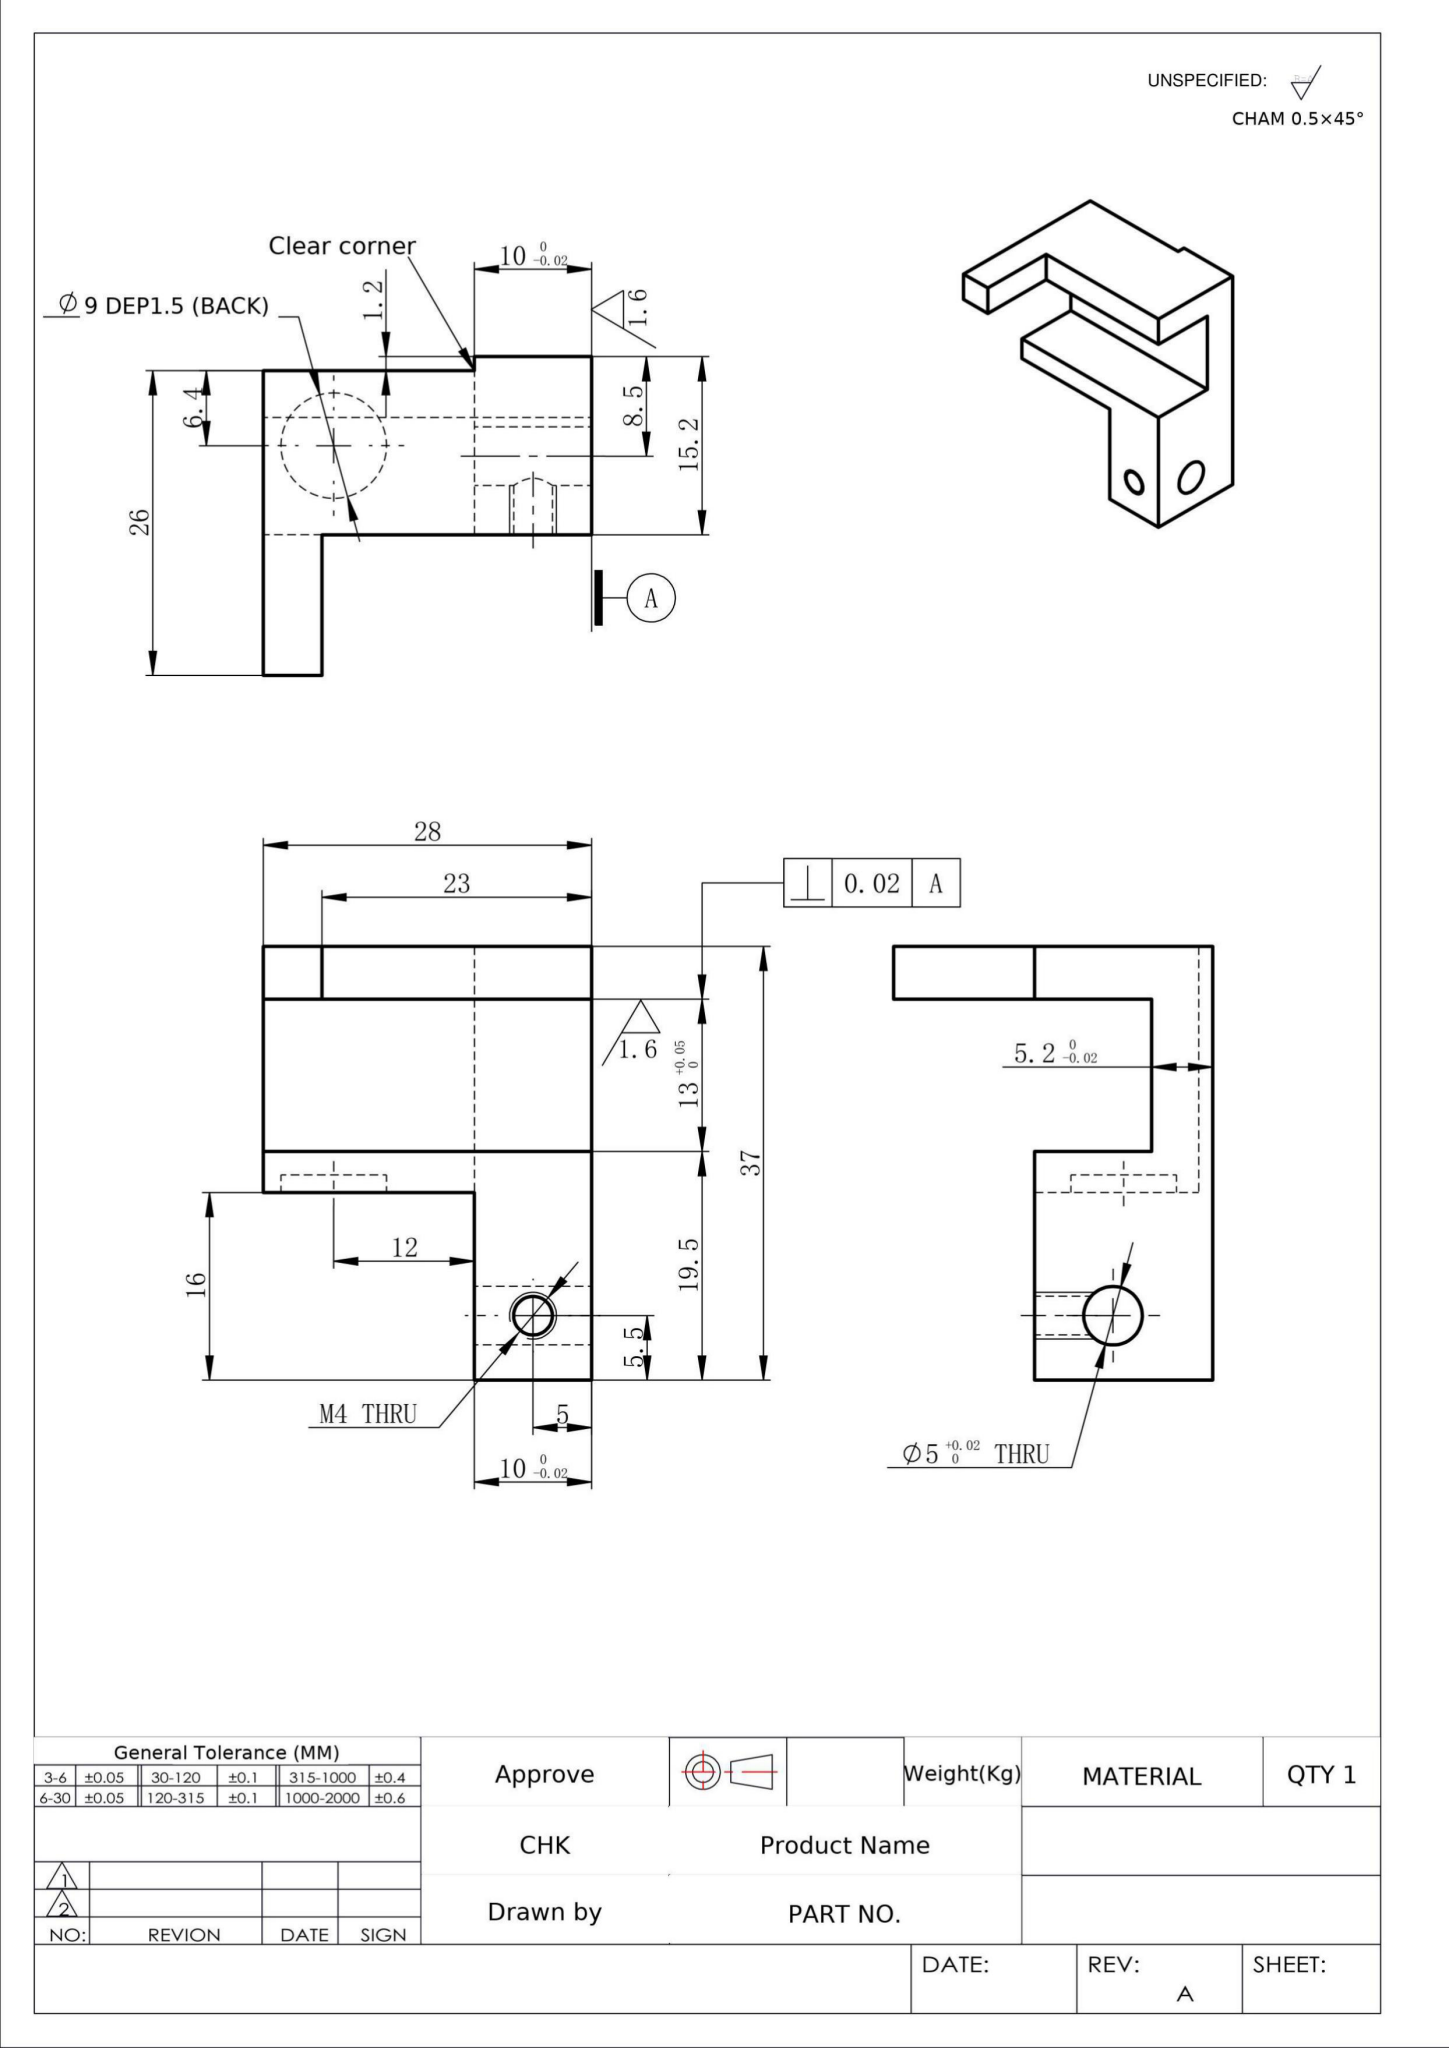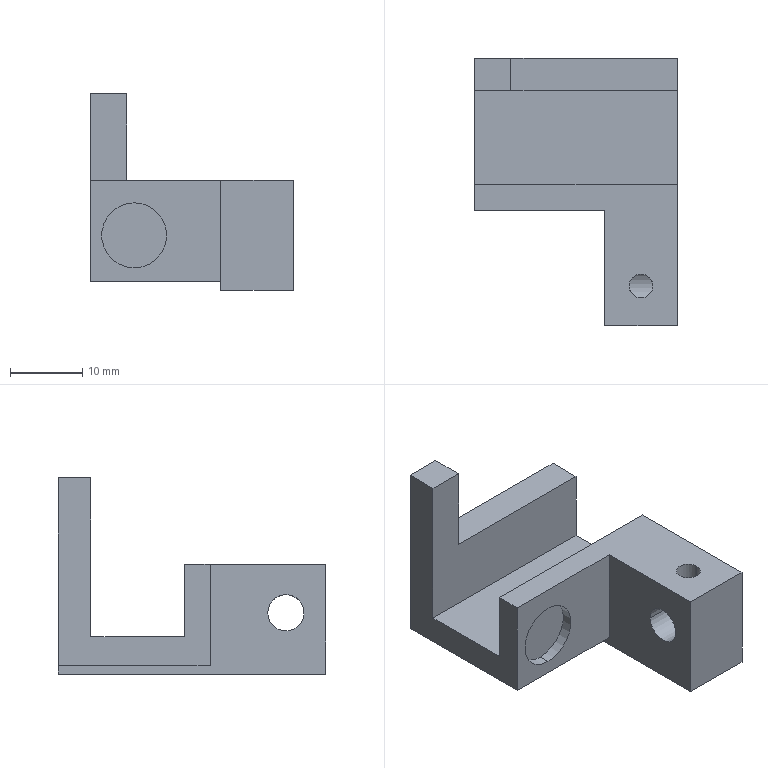Part | NX | mm | Offset Slide Clamp Block | 1 solid | 22 faces | box 28 x 37 x 27.2 mm | volume 7217 mm3 | plane 16 | cylinder 6 | commonest cylinder face diameters 3.3 x2 5 x2 9 x2
STEP:
#1=COLOUR_RGB('',0.7961,0.8235,0.9373);
#2=FILL_AREA_STYLE_COLOUR('',#1);
#3=FILL_AREA_STYLE('',(#2));
#4=SURFACE_STYLE_FILL_AREA(#3);
#5=SURFACE_SIDE_STYLE('',(#4));
#6=SURFACE_STYLE_USAGE(.BOTH.,#5);
#7=PRESENTATION_STYLE_ASSIGNMENT((#6));
#8=CARTESIAN_POINT('',(-6.65,-31.5,11.));
#9=VERTEX_POINT('',#8);
#10=CARTESIAN_POINT('',(-3.35,-31.5,11.));
#11=VERTEX_POINT('',#10);
#12=CARTESIAN_POINT('',(-6.65,-31.5,11.));
#13=CARTESIAN_POINT('',(-6.65,-31.611,11.));
#14=CARTESIAN_POINT('',(-6.639,-31.724,10.992));
#15=CARTESIAN_POINT('',(-6.594,-31.941,10.963));
#16=CARTESIAN_POINT('',(-6.561,-32.045,10.942));
#17=CARTESIAN_POINT('',(-6.433,-32.346,10.862));
#18=CARTESIAN_POINT('',(-6.311,-32.524,10.787));
#19=CARTESIAN_POINT('',(-6.088,-32.745,10.67));
#20=CARTESIAN_POINT('',(-6.008,-32.811,10.63));
#21=CARTESIAN_POINT('',(-5.834,-32.928,10.553));
#22=CARTESIAN_POINT('',(-5.74,-32.979,10.516));
#23=CARTESIAN_POINT('',(-5.445,-33.103,10.421));
#24=CARTESIAN_POINT('',(-5.224,-33.15,10.378));
#25=CARTESIAN_POINT('',(-4.775,-33.15,10.378));
#26=CARTESIAN_POINT('',(-4.553,-33.102,10.422));
#27=CARTESIAN_POINT('',(-4.16,-32.936,10.549));
#28=CARTESIAN_POINT('',(-3.984,-32.816,10.632));
#29=CARTESIAN_POINT('',(-3.688,-32.522,10.788));
#30=CARTESIAN_POINT('',(-3.566,-32.344,10.862));
#31=CARTESIAN_POINT('',(-3.44,-32.047,10.942));
#32=CARTESIAN_POINT('',(-3.406,-31.941,10.963));
#33=CARTESIAN_POINT('',(-3.361,-31.724,10.992));
#34=CARTESIAN_POINT('',(-3.35,-31.613,11.));
#35=CARTESIAN_POINT('',(-3.35,-31.5,11.));
#36=B_SPLINE_CURVE_WITH_KNOTS('',3,(#12,#13,#14,#15,#16,#17,#18,#19,#20,#21,#22,#23,#24,#25,#26,#27,#28,#29,#30,#31,#32,#33,#34,#35),.UNSPECIFIED.,.F.,.F.,(4,2,2,2,2,2,2,2,2,2,2,4),(0.005328,0.005661,0.005993,0.006658,0.006991,0.007324,0.007989,0.008654,0.009319,0.009984,0.01032,0.01065),.UNSPECIFIED.);
#37=EDGE_CURVE('',#9,#11,#36,.T.);
#38=ORIENTED_EDGE('',*,*,#37,.F.);
#39=CARTESIAN_POINT('',(-6.65,-31.5,15.2));
#40=VERTEX_POINT('',#39);
#41=CARTESIAN_POINT('',(-6.65,-31.5,15.2));
#42=DIRECTION('',(0.,0.,1.));
#43=VECTOR('',#42,1000.);
#44=LINE('',#41,#43);
#45=EDGE_CURVE('',#9,#40,#44,.T.);
#46=ORIENTED_EDGE('',*,*,#45,.T.);
#47=CARTESIAN_POINT('',(-3.35,-31.5,15.2));
#48=VERTEX_POINT('',#47);
#49=CARTESIAN_POINT('',(-5.,-31.5,15.2));
#50=DIRECTION('',(0.,0.,1.));
#51=DIRECTION('',(1.,0.,0.));
#52=AXIS2_PLACEMENT_3D('',#49,#50,#51);
#53=CIRCLE('',#52,1.65);
#54=EDGE_CURVE('',#40,#48,#53,.T.);
#55=ORIENTED_EDGE('',*,*,#54,.T.);
#56=CARTESIAN_POINT('',(-3.35,-31.5,15.2));
#57=DIRECTION('',(0.,0.,1.));
#58=VECTOR('',#57,1000.);
#59=LINE('',#56,#58);
#60=EDGE_CURVE('',#11,#48,#59,.T.);
#61=ORIENTED_EDGE('',*,*,#60,.F.);
#62=EDGE_LOOP('',(#38,#46,#55,#61));
#63=FACE_OUTER_BOUND('',#62,.T.);
#64=CARTESIAN_POINT('',(-5.,-31.5,15.2));
#65=DIRECTION('',(0.,0.,1.));
#66=DIRECTION('',(1.,0.,0.));
#67=AXIS2_PLACEMENT_3D('',#64,#65,#66);
#68=CYLINDRICAL_SURFACE('',#67,1.65);
#69=ADVANCED_FACE('',(#63),#68,.F.);
#70=CARTESIAN_POINT('',(-10.,-34.,8.5));
#71=VERTEX_POINT('',#70);
#72=CARTESIAN_POINT('',(-10.,-29.,8.5));
#73=VERTEX_POINT('',#72);
#74=CARTESIAN_POINT('',(-10.,-31.5,8.5));
#75=DIRECTION('',(1.,0.,0.));
#76=DIRECTION('',(0.,1.,0.));
#77=AXIS2_PLACEMENT_3D('',#74,#75,#76);
#78=CIRCLE('',#77,2.5);
#79=EDGE_CURVE('',#71,#73,#78,.T.);
#80=ORIENTED_EDGE('',*,*,#79,.F.);
#81=CARTESIAN_POINT('',(0.,-34.,8.5));
#82=VERTEX_POINT('',#81);
#83=CARTESIAN_POINT('',(-28.,-34.,8.5));
#84=DIRECTION('',(1.,0.,0.));
#85=VECTOR('',#84,1000.);
#86=LINE('',#83,#85);
#87=EDGE_CURVE('',#71,#82,#86,.T.);
#88=ORIENTED_EDGE('',*,*,#87,.T.);
#89=CARTESIAN_POINT('',(0.,-29.,8.5));
#90=VERTEX_POINT('',#89);
#91=CARTESIAN_POINT('',(0.,-31.5,8.5));
#92=DIRECTION('',(1.,0.,0.));
#93=DIRECTION('',(-0.,1.,0.));
#94=AXIS2_PLACEMENT_3D('',#91,#92,#93);
#95=CIRCLE('',#94,2.5);
#96=EDGE_CURVE('',#82,#90,#95,.T.);
#97=ORIENTED_EDGE('',*,*,#96,.T.);
#98=CARTESIAN_POINT('',(-28.,-29.,8.5));
#99=DIRECTION('',(1.,0.,0.));
#100=VECTOR('',#99,1000.);
#101=LINE('',#98,#100);
#102=EDGE_CURVE('',#73,#90,#101,.T.);
#103=ORIENTED_EDGE('',*,*,#102,.F.);
#104=EDGE_LOOP('',(#80,#88,#97,#103));
#105=FACE_OUTER_BOUND('',#104,.T.);
#106=CARTESIAN_POINT('',(-28.,-31.5,8.5));
#107=DIRECTION('',(1.,0.,0.));
#108=DIRECTION('',(0.,1.,0.));
#109=AXIS2_PLACEMENT_3D('',#106,#107,#108);
#110=CYLINDRICAL_SURFACE('',#109,2.5);
#111=ADVANCED_FACE('',(#105),#110,.F.);
#112=CARTESIAN_POINT('',(-22.,-19.5,12.1));
#113=VERTEX_POINT('',#112);
#114=CARTESIAN_POINT('',(-22.,-19.5,3.1));
#115=VERTEX_POINT('',#114);
#116=CARTESIAN_POINT('',(-22.,-19.5,7.6));
#117=DIRECTION('',(0.,-1.,0.));
#118=DIRECTION('',(0.,0.,-1.));
#119=AXIS2_PLACEMENT_3D('',#116,#117,#118);
#120=CIRCLE('',#119,4.5);
#121=EDGE_CURVE('',#113,#115,#120,.T.);
#122=ORIENTED_EDGE('',*,*,#121,.F.);
#123=CARTESIAN_POINT('',(-22.,-21.,12.1));
#124=VERTEX_POINT('',#123);
#125=CARTESIAN_POINT('',(-22.,-19.5,12.1));
#126=DIRECTION('',(0.,-1.,0.));
#127=VECTOR('',#126,1000.);
#128=LINE('',#125,#127);
#129=EDGE_CURVE('',#113,#124,#128,.T.);
#130=ORIENTED_EDGE('',*,*,#129,.T.);
#131=CARTESIAN_POINT('',(-22.,-21.,3.1));
#132=VERTEX_POINT('',#131);
#133=CARTESIAN_POINT('',(-22.,-21.,7.6));
#134=DIRECTION('',(0.,-1.,0.));
#135=DIRECTION('',(0.,0.,-1.));
#136=AXIS2_PLACEMENT_3D('',#133,#134,#135);
#137=CIRCLE('',#136,4.5);
#138=EDGE_CURVE('',#124,#132,#137,.T.);
#139=ORIENTED_EDGE('',*,*,#138,.T.);
#140=CARTESIAN_POINT('',(-22.,-19.5,3.1));
#141=DIRECTION('',(0.,-1.,0.));
#142=VECTOR('',#141,1000.);
#143=LINE('',#140,#142);
#144=EDGE_CURVE('',#115,#132,#143,.T.);
#145=ORIENTED_EDGE('',*,*,#144,.F.);
#146=EDGE_LOOP('',(#122,#130,#139,#145));
#147=FACE_OUTER_BOUND('',#146,.T.);
#148=CARTESIAN_POINT('',(-22.,-19.5,7.6));
#149=DIRECTION('',(0.,-1.,0.));
#150=DIRECTION('',(0.,0.,-1.));
#151=AXIS2_PLACEMENT_3D('',#148,#149,#150);
#152=CYLINDRICAL_SURFACE('',#151,4.5);
#153=ADVANCED_FACE('',(#147),#152,.F.);
#154=CARTESIAN_POINT('',(-23.,0.,15.2));
#155=VERTEX_POINT('',#154);
#156=CARTESIAN_POINT('',(-23.,-4.5,15.2));
#157=VERTEX_POINT('',#156);
#158=CARTESIAN_POINT('',(-23.,-4.5,15.2));
#159=DIRECTION('',(0.,-1.,0.));
#160=VECTOR('',#159,1000.);
#161=LINE('',#158,#160);
#162=EDGE_CURVE('',#155,#157,#161,.T.);
#163=ORIENTED_EDGE('',*,*,#162,.T.);
#164=CARTESIAN_POINT('',(0.,-4.5,15.2));
#165=VERTEX_POINT('',#164);
#166=CARTESIAN_POINT('',(-28.,-4.5,15.2));
#167=DIRECTION('',(-1.,0.,0.));
#168=VECTOR('',#167,1000.);
#169=LINE('',#166,#168);
#170=EDGE_CURVE('',#165,#157,#169,.T.);
#171=ORIENTED_EDGE('',*,*,#170,.F.);
#172=CARTESIAN_POINT('',(0.,0.,15.2));
#173=VERTEX_POINT('',#172);
#174=CARTESIAN_POINT('',(0.,0.,15.2));
#175=DIRECTION('',(-0.,1.,0.));
#176=VECTOR('',#175,1000.);
#177=LINE('',#174,#176);
#178=EDGE_CURVE('',#165,#173,#177,.T.);
#179=ORIENTED_EDGE('',*,*,#178,.T.);
#180=CARTESIAN_POINT('',(-23.,0.,15.2));
#181=DIRECTION('',(-1.,0.,0.));
#182=VECTOR('',#181,1000.);
#183=LINE('',#180,#182);
#184=EDGE_CURVE('',#173,#155,#183,.T.);
#185=ORIENTED_EDGE('',*,*,#184,.T.);
#186=EDGE_LOOP('',(#163,#171,#179,#185));
#187=FACE_OUTER_BOUND('',#186,.T.);
#188=CARTESIAN_POINT('',(-28.,-4.5,15.2));
#189=DIRECTION('',(0.,0.,-1.));
#190=DIRECTION('',(-1.,0.,0.));
#191=AXIS2_PLACEMENT_3D('',#188,#189,#190);
#192=PLANE('',#191);
#193=ADVANCED_FACE('',(#187),#192,.F.);
#194=CARTESIAN_POINT('',(0.,-31.5,8.5));
#195=DIRECTION('',(1.,0.,0.));
#196=DIRECTION('',(-0.,1.,0.));
#197=AXIS2_PLACEMENT_3D('',#194,#195,#196);
#198=CIRCLE('',#197,2.5);
#199=EDGE_CURVE('',#90,#82,#198,.T.);
#200=ORIENTED_EDGE('',*,*,#199,.F.);
#201=ORIENTED_EDGE('',*,*,#96,.F.);
#202=EDGE_LOOP('',(#200,#201));
#203=FACE_BOUND('',#202,.T.);
#204=ORIENTED_EDGE('',*,*,#178,.F.);
#205=CARTESIAN_POINT('',(0.,-4.5,5.2));
#206=VERTEX_POINT('',#205);
#207=CARTESIAN_POINT('',(0.,-4.5,5.2));
#208=DIRECTION('',(0.,0.,1.));
#209=VECTOR('',#208,1000.);
#210=LINE('',#207,#209);
#211=EDGE_CURVE('',#206,#165,#210,.T.);
#212=ORIENTED_EDGE('',*,*,#211,.F.);
#213=CARTESIAN_POINT('',(0.,-17.5,5.2));
#214=VERTEX_POINT('',#213);
#215=CARTESIAN_POINT('',(0.,-4.5,5.2));
#216=DIRECTION('',(-0.,1.,0.));
#217=VECTOR('',#216,1000.);
#218=LINE('',#215,#217);
#219=EDGE_CURVE('',#214,#206,#218,.T.);
#220=ORIENTED_EDGE('',*,*,#219,.F.);
#221=CARTESIAN_POINT('',(0.,-17.5,15.2));
#222=VERTEX_POINT('',#221);
#223=CARTESIAN_POINT('',(0.,-17.5,5.2));
#224=DIRECTION('',(0.,0.,1.));
#225=VECTOR('',#224,1000.);
#226=LINE('',#223,#225);
#227=EDGE_CURVE('',#214,#222,#226,.T.);
#228=ORIENTED_EDGE('',*,*,#227,.T.);
#229=CARTESIAN_POINT('',(0.,-37.,15.2));
#230=VERTEX_POINT('',#229);
#231=CARTESIAN_POINT('',(0.,0.,15.2));
#232=DIRECTION('',(-0.,1.,0.));
#233=VECTOR('',#232,1000.);
#234=LINE('',#231,#233);
#235=EDGE_CURVE('',#230,#222,#234,.T.);
#236=ORIENTED_EDGE('',*,*,#235,.F.);
#237=CARTESIAN_POINT('',(0.,-37.,0.));
#238=VERTEX_POINT('',#237);
#239=CARTESIAN_POINT('',(0.,-37.,27.2));
#240=DIRECTION('',(0.,0.,-1.));
#241=VECTOR('',#240,1000.);
#242=LINE('',#239,#241);
#243=EDGE_CURVE('',#230,#238,#242,.T.);
#244=ORIENTED_EDGE('',*,*,#243,.T.);
#245=CARTESIAN_POINT('',(0.,0.,0.));
#246=VERTEX_POINT('',#245);
#247=CARTESIAN_POINT('',(0.,0.,0.));
#248=DIRECTION('',(-0.,1.,0.));
#249=VECTOR('',#248,1000.);
#250=LINE('',#247,#249);
#251=EDGE_CURVE('',#238,#246,#250,.T.);
#252=ORIENTED_EDGE('',*,*,#251,.T.);
#253=CARTESIAN_POINT('',(0.,0.,27.2));
#254=DIRECTION('',(0.,0.,-1.));
#255=VECTOR('',#254,1000.);
#256=LINE('',#253,#255);
#257=EDGE_CURVE('',#173,#246,#256,.T.);
#258=ORIENTED_EDGE('',*,*,#257,.F.);
#259=EDGE_LOOP('',(#204,#212,#220,#228,#236,#244,#252,#258));
#260=FACE_OUTER_BOUND('',#259,.T.);
#261=CARTESIAN_POINT('',(0.,0.,27.2));
#262=DIRECTION('',(-1.,-0.,0.));
#263=DIRECTION('',(0.,-1.,0.));
#264=AXIS2_PLACEMENT_3D('',#261,#262,#263);
#265=PLANE('',#264);
#266=ADVANCED_FACE('',(#203,#260),#265,.F.);
#267=CARTESIAN_POINT('',(-10.,-0.,0.));
#268=VERTEX_POINT('',#267);
#269=CARTESIAN_POINT('',(0.,0.,0.));
#270=DIRECTION('',(-1.,-0.,0.));
#271=VECTOR('',#270,1000.);
#272=LINE('',#269,#271);
#273=EDGE_CURVE('',#246,#268,#272,.T.);
#274=ORIENTED_EDGE('',*,*,#273,.T.);
#275=CARTESIAN_POINT('',(-10.,-0.,1.2));
#276=VERTEX_POINT('',#275);
#277=CARTESIAN_POINT('',(-10.,-0.,1.2));
#278=DIRECTION('',(0.,0.,-1.));
#279=VECTOR('',#278,1000.);
#280=LINE('',#277,#279);
#281=EDGE_CURVE('',#276,#268,#280,.T.);
#282=ORIENTED_EDGE('',*,*,#281,.F.);
#283=CARTESIAN_POINT('',(-28.,-0.,1.2));
#284=VERTEX_POINT('',#283);
#285=CARTESIAN_POINT('',(-10.,-0.,1.2));
#286=DIRECTION('',(1.,0.,0.));
#287=VECTOR('',#286,1000.);
#288=LINE('',#285,#287);
#289=EDGE_CURVE('',#284,#276,#288,.T.);
#290=ORIENTED_EDGE('',*,*,#289,.F.);
#291=CARTESIAN_POINT('',(-28.,-0.,27.2));
#292=VERTEX_POINT('',#291);
#293=CARTESIAN_POINT('',(-28.,-0.,27.2));
#294=DIRECTION('',(0.,0.,-1.));
#295=VECTOR('',#294,1000.);
#296=LINE('',#293,#295);
#297=EDGE_CURVE('',#292,#284,#296,.T.);
#298=ORIENTED_EDGE('',*,*,#297,.F.);
#299=CARTESIAN_POINT('',(-23.,-0.,27.2));
#300=VERTEX_POINT('',#299);
#301=CARTESIAN_POINT('',(0.,0.,27.2));
#302=DIRECTION('',(-1.,-0.,0.));
#303=VECTOR('',#302,1000.);
#304=LINE('',#301,#303);
#305=EDGE_CURVE('',#300,#292,#304,.T.);
#306=ORIENTED_EDGE('',*,*,#305,.F.);
#307=CARTESIAN_POINT('',(-23.,0.,15.2));
#308=DIRECTION('',(0.,0.,1.));
#309=VECTOR('',#308,1000.);
#310=LINE('',#307,#309);
#311=EDGE_CURVE('',#155,#300,#310,.T.);
#312=ORIENTED_EDGE('',*,*,#311,.F.);
#313=ORIENTED_EDGE('',*,*,#184,.F.);
#314=ORIENTED_EDGE('',*,*,#257,.T.);
#315=EDGE_LOOP('',(#274,#282,#290,#298,#306,#312,#313,#314));
#316=FACE_OUTER_BOUND('',#315,.T.);
#317=CARTESIAN_POINT('',(0.,0.,27.2));
#318=DIRECTION('',(0.,-1.,0.));
#319=DIRECTION('',(1.,0.,0.));
#320=AXIS2_PLACEMENT_3D('',#317,#318,#319);
#321=PLANE('',#320);
#322=ADVANCED_FACE('',(#316),#321,.F.);
#323=ORIENTED_EDGE('',*,*,#297,.T.);
#324=CARTESIAN_POINT('',(-28.,-21.,1.2));
#325=VERTEX_POINT('',#324);
#326=CARTESIAN_POINT('',(-28.,-21.,1.2));
#327=DIRECTION('',(0.,1.,0.));
#328=VECTOR('',#327,1000.);
#329=LINE('',#326,#328);
#330=EDGE_CURVE('',#325,#284,#329,.T.);
#331=ORIENTED_EDGE('',*,*,#330,.F.);
#332=CARTESIAN_POINT('',(-28.,-21.,15.2));
#333=VERTEX_POINT('',#332);
#334=CARTESIAN_POINT('',(-28.,-21.,27.2));
#335=DIRECTION('',(0.,0.,-1.));
#336=VECTOR('',#335,1000.);
#337=LINE('',#334,#336);
#338=EDGE_CURVE('',#333,#325,#337,.T.);
#339=ORIENTED_EDGE('',*,*,#338,.F.);
#340=CARTESIAN_POINT('',(-28.,-17.5,15.2));
#341=VERTEX_POINT('',#340);
#342=CARTESIAN_POINT('',(-28.,-21.,15.2));
#343=DIRECTION('',(0.,-1.,0.));
#344=VECTOR('',#343,1000.);
#345=LINE('',#342,#344);
#346=EDGE_CURVE('',#341,#333,#345,.T.);
#347=ORIENTED_EDGE('',*,*,#346,.F.);
#348=CARTESIAN_POINT('',(-28.,-17.5,5.2));
#349=VERTEX_POINT('',#348);
#350=CARTESIAN_POINT('',(-28.,-17.5,5.2));
#351=DIRECTION('',(0.,0.,1.));
#352=VECTOR('',#351,1000.);
#353=LINE('',#350,#352);
#354=EDGE_CURVE('',#349,#341,#353,.T.);
#355=ORIENTED_EDGE('',*,*,#354,.F.);
#356=CARTESIAN_POINT('',(-28.,-4.5,5.2));
#357=VERTEX_POINT('',#356);
#358=CARTESIAN_POINT('',(-28.,-4.5,5.2));
#359=DIRECTION('',(0.,-1.,0.));
#360=VECTOR('',#359,1000.);
#361=LINE('',#358,#360);
#362=EDGE_CURVE('',#357,#349,#361,.T.);
#363=ORIENTED_EDGE('',*,*,#362,.F.);
#364=CARTESIAN_POINT('',(-28.,-4.5,27.2));
#365=VERTEX_POINT('',#364);
#366=CARTESIAN_POINT('',(-28.,-4.5,15.2));
#367=DIRECTION('',(0.,0.,1.));
#368=VECTOR('',#367,1000.);
#369=LINE('',#366,#368);
#370=EDGE_CURVE('',#357,#365,#369,.T.);
#371=ORIENTED_EDGE('',*,*,#370,.T.);
#372=CARTESIAN_POINT('',(-28.,-0.,27.2));
#373=DIRECTION('',(0.,-1.,0.));
#374=VECTOR('',#373,1000.);
#375=LINE('',#372,#374);
#376=EDGE_CURVE('',#292,#365,#375,.T.);
#377=ORIENTED_EDGE('',*,*,#376,.F.);
#378=EDGE_LOOP('',(#323,#331,#339,#347,#355,#363,#371,#377));
#379=FACE_OUTER_BOUND('',#378,.T.);
#380=CARTESIAN_POINT('',(-28.,-0.,27.2));
#381=DIRECTION('',(1.,0.,0.));
#382=DIRECTION('',(0.,0.,-1.));
#383=AXIS2_PLACEMENT_3D('',#380,#381,#382);
#384=PLANE('',#383);
#385=ADVANCED_FACE('',(#379),#384,.F.);
#386=CARTESIAN_POINT('',(-22.,-21.,7.6));
#387=DIRECTION('',(0.,-1.,0.));
#388=DIRECTION('',(0.,0.,-1.));
#389=AXIS2_PLACEMENT_3D('',#386,#387,#388);
#390=CIRCLE('',#389,4.5);
#391=EDGE_CURVE('',#132,#124,#390,.T.);
#392=ORIENTED_EDGE('',*,*,#391,.F.);
#393=ORIENTED_EDGE('',*,*,#138,.F.);
#394=EDGE_LOOP('',(#392,#393));
#395=FACE_BOUND('',#394,.T.);
#396=ORIENTED_EDGE('',*,*,#338,.T.);
#397=CARTESIAN_POINT('',(-10.,-21.,1.2));
#398=VERTEX_POINT('',#397);
#399=CARTESIAN_POINT('',(-10.,-21.,1.2));
#400=DIRECTION('',(-1.,0.,0.));
#401=VECTOR('',#400,1000.);
#402=LINE('',#399,#401);
#403=EDGE_CURVE('',#398,#325,#402,.T.);
#404=ORIENTED_EDGE('',*,*,#403,.F.);
#405=CARTESIAN_POINT('',(-10.,-21.,15.2));
#406=VERTEX_POINT('',#405);
#407=CARTESIAN_POINT('',(-10.,-21.,27.2));
#408=DIRECTION('',(0.,0.,-1.));
#409=VECTOR('',#408,1000.);
#410=LINE('',#407,#409);
#411=EDGE_CURVE('',#406,#398,#410,.T.);
#412=ORIENTED_EDGE('',*,*,#411,.F.);
#413=CARTESIAN_POINT('',(-10.,-21.,15.2));
#414=DIRECTION('',(1.,0.,0.));
#415=VECTOR('',#414,1000.);
#416=LINE('',#413,#415);
#417=EDGE_CURVE('',#333,#406,#416,.T.);
#418=ORIENTED_EDGE('',*,*,#417,.F.);
#419=EDGE_LOOP('',(#396,#404,#412,#418));
#420=FACE_OUTER_BOUND('',#419,.T.);
#421=CARTESIAN_POINT('',(-28.,-21.,27.2));
#422=DIRECTION('',(0.,1.,0.));
#423=DIRECTION('',(0.,0.,1.));
#424=AXIS2_PLACEMENT_3D('',#421,#422,#423);
#425=PLANE('',#424);
#426=ADVANCED_FACE('',(#395,#420),#425,.F.);
#427=CARTESIAN_POINT('',(-10.,-31.5,8.5));
#428=DIRECTION('',(1.,0.,0.));
#429=DIRECTION('',(0.,1.,0.));
#430=AXIS2_PLACEMENT_3D('',#427,#428,#429);
#431=CIRCLE('',#430,2.5);
#432=EDGE_CURVE('',#73,#71,#431,.T.);
#433=ORIENTED_EDGE('',*,*,#432,.T.);
#434=ORIENTED_EDGE('',*,*,#79,.T.);
#435=EDGE_LOOP('',(#433,#434));
#436=FACE_BOUND('',#435,.T.);
#437=CARTESIAN_POINT('',(-10.,-37.,15.2));
#438=VERTEX_POINT('',#437);
#439=CARTESIAN_POINT('',(-10.,-37.,0.));
#440=VERTEX_POINT('',#439);
#441=CARTESIAN_POINT('',(-10.,-37.,27.2));
#442=DIRECTION('',(0.,0.,-1.));
#443=VECTOR('',#442,1000.);
#444=LINE('',#441,#443);
#445=EDGE_CURVE('',#438,#440,#444,.T.);
#446=ORIENTED_EDGE('',*,*,#445,.F.);
#447=CARTESIAN_POINT('',(-10.,-37.,15.2));
#448=DIRECTION('',(0.,-1.,0.));
#449=VECTOR('',#448,1000.);
#450=LINE('',#447,#449);
#451=EDGE_CURVE('',#406,#438,#450,.T.);
#452=ORIENTED_EDGE('',*,*,#451,.F.);
#453=ORIENTED_EDGE('',*,*,#411,.T.);
#454=CARTESIAN_POINT('',(-10.,-21.,1.2));
#455=DIRECTION('',(0.,-1.,0.));
#456=VECTOR('',#455,1000.);
#457=LINE('',#454,#456);
#458=EDGE_CURVE('',#276,#398,#457,.T.);
#459=ORIENTED_EDGE('',*,*,#458,.F.);
#460=ORIENTED_EDGE('',*,*,#281,.T.);
#461=CARTESIAN_POINT('',(-10.,-21.,0.));
#462=DIRECTION('',(0.,-1.,0.));
#463=VECTOR('',#462,1000.);
#464=LINE('',#461,#463);
#465=EDGE_CURVE('',#268,#440,#464,.T.);
#466=ORIENTED_EDGE('',*,*,#465,.T.);
#467=EDGE_LOOP('',(#446,#452,#453,#459,#460,#466));
#468=FACE_OUTER_BOUND('',#467,.T.);
#469=CARTESIAN_POINT('',(-10.,-21.,27.2));
#470=DIRECTION('',(1.,0.,0.));
#471=DIRECTION('',(-0.,1.,0.));
#472=AXIS2_PLACEMENT_3D('',#469,#470,#471);
#473=PLANE('',#472);
#474=ADVANCED_FACE('',(#436,#468),#473,.F.);
#475=ORIENTED_EDGE('',*,*,#243,.F.);
#476=CARTESIAN_POINT('',(0.,-37.,15.2));
#477=DIRECTION('',(1.,0.,0.));
#478=VECTOR('',#477,1000.);
#479=LINE('',#476,#478);
#480=EDGE_CURVE('',#438,#230,#479,.T.);
#481=ORIENTED_EDGE('',*,*,#480,.F.);
#482=ORIENTED_EDGE('',*,*,#445,.T.);
#483=CARTESIAN_POINT('',(-10.,-37.,0.));
#484=DIRECTION('',(1.,0.,0.));
#485=VECTOR('',#484,1000.);
#486=LINE('',#483,#485);
#487=EDGE_CURVE('',#440,#238,#486,.T.);
#488=ORIENTED_EDGE('',*,*,#487,.T.);
#489=EDGE_LOOP('',(#475,#481,#482,#488));
#490=FACE_OUTER_BOUND('',#489,.T.);
#491=CARTESIAN_POINT('',(-10.,-37.,27.2));
#492=DIRECTION('',(0.,1.,0.));
#493=DIRECTION('',(0.,0.,1.));
#494=AXIS2_PLACEMENT_3D('',#491,#492,#493);
#495=PLANE('',#494);
#496=ADVANCED_FACE('',(#490),#495,.F.);
#497=CARTESIAN_POINT('',(-23.,-4.5,27.2));
#498=VERTEX_POINT('',#497);
#499=CARTESIAN_POINT('',(-28.,-4.5,27.2));
#500=DIRECTION('',(-1.,0.,0.));
#501=VECTOR('',#500,1000.);
#502=LINE('',#499,#501);
#503=EDGE_CURVE('',#498,#365,#502,.T.);
#504=ORIENTED_EDGE('',*,*,#503,.F.);
#505=CARTESIAN_POINT('',(-23.,-4.5,27.2));
#506=DIRECTION('',(0.,-1.,0.));
#507=VECTOR('',#506,1000.);
#508=LINE('',#505,#507);
#509=EDGE_CURVE('',#300,#498,#508,.T.);
#510=ORIENTED_EDGE('',*,*,#509,.F.);
#511=ORIENTED_EDGE('',*,*,#305,.T.);
#512=ORIENTED_EDGE('',*,*,#376,.T.);
#513=EDGE_LOOP('',(#504,#510,#511,#512));
#514=FACE_OUTER_BOUND('',#513,.T.);
#515=CARTESIAN_POINT('',(0.,-37.,27.2));
#516=DIRECTION('',(0.,0.,1.));
#517=DIRECTION('',(1.,0.,0.));
#518=AXIS2_PLACEMENT_3D('',#515,#516,#517);
#519=PLANE('',#518);
#520=ADVANCED_FACE('',(#514),#519,.T.);
#521=ORIENTED_EDGE('',*,*,#465,.F.);
#522=ORIENTED_EDGE('',*,*,#273,.F.);
#523=ORIENTED_EDGE('',*,*,#251,.F.);
#524=ORIENTED_EDGE('',*,*,#487,.F.);
#525=EDGE_LOOP('',(#521,#522,#523,#524));
#526=FACE_OUTER_BOUND('',#525,.T.);
#527=CARTESIAN_POINT('',(0.,-37.,0.));
#528=DIRECTION('',(0.,0.,1.));
#529=DIRECTION('',(1.,0.,0.));
#530=AXIS2_PLACEMENT_3D('',#527,#528,#529);
#531=PLANE('',#530);
#532=ADVANCED_FACE('',(#526),#531,.F.);
#533=ORIENTED_EDGE('',*,*,#503,.T.);
#534=ORIENTED_EDGE('',*,*,#370,.F.);
#535=CARTESIAN_POINT('',(-28.,-4.5,5.2));
#536=DIRECTION('',(-1.,0.,0.));
#537=VECTOR('',#536,1000.);
#538=LINE('',#535,#537);
#539=EDGE_CURVE('',#206,#357,#538,.T.);
#540=ORIENTED_EDGE('',*,*,#539,.F.);
#541=ORIENTED_EDGE('',*,*,#211,.T.);
#542=ORIENTED_EDGE('',*,*,#170,.T.);
#543=CARTESIAN_POINT('',(-23.,-4.5,15.2));
#544=DIRECTION('',(0.,0.,1.));
#545=VECTOR('',#544,1000.);
#546=LINE('',#543,#545);
#547=EDGE_CURVE('',#157,#498,#546,.T.);
#548=ORIENTED_EDGE('',*,*,#547,.T.);
#549=EDGE_LOOP('',(#533,#534,#540,#541,#542,#548));
#550=FACE_OUTER_BOUND('',#549,.T.);
#551=CARTESIAN_POINT('',(-28.,-4.5,15.2));
#552=DIRECTION('',(0.,1.,0.));
#553=DIRECTION('',(0.,0.,1.));
#554=AXIS2_PLACEMENT_3D('',#551,#552,#553);
#555=PLANE('',#554);
#556=ADVANCED_FACE('',(#550),#555,.F.);
#557=ORIENTED_EDGE('',*,*,#509,.T.);
#558=ORIENTED_EDGE('',*,*,#547,.F.);
#559=ORIENTED_EDGE('',*,*,#162,.F.);
#560=ORIENTED_EDGE('',*,*,#311,.T.);
#561=EDGE_LOOP('',(#557,#558,#559,#560));
#562=FACE_OUTER_BOUND('',#561,.T.);
#563=CARTESIAN_POINT('',(-23.,-4.5,15.2));
#564=DIRECTION('',(-1.,0.,0.));
#565=DIRECTION('',(0.,0.,1.));
#566=AXIS2_PLACEMENT_3D('',#563,#564,#565);
#567=PLANE('',#566);
#568=ADVANCED_FACE('',(#562),#567,.F.);
#569=CARTESIAN_POINT('',(-5.,-31.5,15.2));
#570=DIRECTION('',(0.,0.,1.));
#571=DIRECTION('',(1.,0.,0.));
#572=AXIS2_PLACEMENT_3D('',#569,#570,#571);
#573=CIRCLE('',#572,1.65);
#574=EDGE_CURVE('',#48,#40,#573,.T.);
#575=ORIENTED_EDGE('',*,*,#574,.F.);
#576=ORIENTED_EDGE('',*,*,#54,.F.);
#577=EDGE_LOOP('',(#575,#576));
#578=FACE_BOUND('',#577,.T.);
#579=ORIENTED_EDGE('',*,*,#235,.T.);
#580=CARTESIAN_POINT('',(-28.,-17.5,15.2));
#581=DIRECTION('',(1.,0.,0.));
#582=VECTOR('',#581,1000.);
#583=LINE('',#580,#582);
#584=EDGE_CURVE('',#341,#222,#583,.T.);
#585=ORIENTED_EDGE('',*,*,#584,.F.);
#586=ORIENTED_EDGE('',*,*,#346,.T.);
#587=ORIENTED_EDGE('',*,*,#417,.T.);
#588=ORIENTED_EDGE('',*,*,#451,.T.);
#589=ORIENTED_EDGE('',*,*,#480,.T.);
#590=EDGE_LOOP('',(#579,#585,#586,#587,#588,#589));
#591=FACE_OUTER_BOUND('',#590,.T.);
#592=CARTESIAN_POINT('',(-28.,-4.5,15.2));
#593=DIRECTION('',(0.,0.,-1.));
#594=DIRECTION('',(-1.,0.,0.));
#595=AXIS2_PLACEMENT_3D('',#592,#593,#594);
#596=PLANE('',#595);
#597=ADVANCED_FACE('',(#578,#591),#596,.F.);
#598=ORIENTED_EDGE('',*,*,#584,.T.);
#599=ORIENTED_EDGE('',*,*,#227,.F.);
#600=CARTESIAN_POINT('',(-28.,-17.5,5.2));
#601=DIRECTION('',(1.,0.,0.));
#602=VECTOR('',#601,1000.);
#603=LINE('',#600,#602);
#604=EDGE_CURVE('',#349,#214,#603,.T.);
#605=ORIENTED_EDGE('',*,*,#604,.F.);
#606=ORIENTED_EDGE('',*,*,#354,.T.);
#607=EDGE_LOOP('',(#598,#599,#605,#606));
#608=FACE_OUTER_BOUND('',#607,.T.);
#609=CARTESIAN_POINT('',(-28.,-17.5,5.2));
#610=DIRECTION('',(0.,-1.,0.));
#611=DIRECTION('',(0.,0.,-1.));
#612=AXIS2_PLACEMENT_3D('',#609,#610,#611);
#613=PLANE('',#612);
#614=ADVANCED_FACE('',(#608),#613,.F.);
#615=ORIENTED_EDGE('',*,*,#362,.T.);
#616=ORIENTED_EDGE('',*,*,#604,.T.);
#617=ORIENTED_EDGE('',*,*,#219,.T.);
#618=ORIENTED_EDGE('',*,*,#539,.T.);
#619=EDGE_LOOP('',(#615,#616,#617,#618));
#620=FACE_OUTER_BOUND('',#619,.T.);
#621=CARTESIAN_POINT('',(-28.,-17.5,5.2));
#622=DIRECTION('',(0.,0.,1.));
#623=DIRECTION('',(1.,0.,0.));
#624=AXIS2_PLACEMENT_3D('',#621,#622,#623);
#625=PLANE('',#624);
#626=ADVANCED_FACE('',(#620),#625,.T.);
#627=ORIENTED_EDGE('',*,*,#129,.F.);
#628=CARTESIAN_POINT('',(-22.,-19.5,7.6));
#629=DIRECTION('',(0.,-1.,0.));
#630=DIRECTION('',(0.,0.,-1.));
#631=AXIS2_PLACEMENT_3D('',#628,#629,#630);
#632=CIRCLE('',#631,4.5);
#633=EDGE_CURVE('',#115,#113,#632,.T.);
#634=ORIENTED_EDGE('',*,*,#633,.F.);
#635=ORIENTED_EDGE('',*,*,#144,.T.);
#636=ORIENTED_EDGE('',*,*,#391,.T.);
#637=EDGE_LOOP('',(#627,#634,#635,#636));
#638=FACE_OUTER_BOUND('',#637,.T.);
#639=CARTESIAN_POINT('',(-22.,-19.5,7.6));
#640=DIRECTION('',(0.,-1.,0.));
#641=DIRECTION('',(0.,0.,-1.));
#642=AXIS2_PLACEMENT_3D('',#639,#640,#641);
#643=CYLINDRICAL_SURFACE('',#642,4.5);
#644=ADVANCED_FACE('',(#638),#643,.F.);
#645=ORIENTED_EDGE('',*,*,#633,.T.);
#646=ORIENTED_EDGE('',*,*,#121,.T.);
#647=EDGE_LOOP('',(#645,#646));
#648=FACE_OUTER_BOUND('',#647,.T.);
#649=CARTESIAN_POINT('',(-22.,-19.5,7.6));
#650=DIRECTION('',(0.,-1.,0.));
#651=DIRECTION('',(0.,0.,-1.));
#652=AXIS2_PLACEMENT_3D('',#649,#650,#651);
#653=PLANE('',#652);
#654=ADVANCED_FACE('',(#648),#653,.T.);
#655=ORIENTED_EDGE('',*,*,#87,.F.);
#656=ORIENTED_EDGE('',*,*,#432,.F.);
#657=ORIENTED_EDGE('',*,*,#102,.T.);
#658=ORIENTED_EDGE('',*,*,#199,.T.);
#659=EDGE_LOOP('',(#655,#656,#657,#658));
#660=FACE_OUTER_BOUND('',#659,.T.);
#661=CARTESIAN_POINT('',(-3.35,-31.5,11.));
#662=CARTESIAN_POINT('',(-3.35,-31.387,11.));
#663=CARTESIAN_POINT('',(-3.361,-31.277,10.992));
#664=CARTESIAN_POINT('',(-3.406,-31.061,10.964));
#665=CARTESIAN_POINT('',(-3.439,-30.954,10.942));
#666=CARTESIAN_POINT('',(-3.566,-30.656,10.862));
#667=CARTESIAN_POINT('',(-3.688,-30.478,10.787));
#668=CARTESIAN_POINT('',(-3.91,-30.257,10.671));
#669=CARTESIAN_POINT('',(-3.992,-30.19,10.63));
#670=CARTESIAN_POINT('',(-4.165,-30.073,10.554));
#671=CARTESIAN_POINT('',(-4.257,-30.023,10.517));
#672=CARTESIAN_POINT('',(-4.552,-29.898,10.422));
#673=CARTESIAN_POINT('',(-4.775,-29.85,10.378));
#674=CARTESIAN_POINT('',(-5.222,-29.85,10.378));
#675=CARTESIAN_POINT('',(-5.443,-29.896,10.421));
#676=CARTESIAN_POINT('',(-5.839,-30.063,10.548));
#677=CARTESIAN_POINT('',(-6.015,-30.182,10.631));
#678=CARTESIAN_POINT('',(-6.238,-30.404,10.749));
#679=CARTESIAN_POINT('',(-6.305,-30.485,10.787));
#680=CARTESIAN_POINT('',(-6.424,-30.659,10.856));
#681=CARTESIAN_POINT('',(-6.476,-30.754,10.888));
#682=CARTESIAN_POINT('',(-6.561,-30.954,10.942));
#683=CARTESIAN_POINT('',(-6.594,-31.059,10.963));
#684=CARTESIAN_POINT('',(-6.639,-31.276,10.992));
#685=CARTESIAN_POINT('',(-6.65,-31.389,11.));
#686=CARTESIAN_POINT('',(-6.65,-31.5,11.));
#687=B_SPLINE_CURVE_WITH_KNOTS('',3,(#661,#662,#663,#664,#665,#666,#667,#668,#669,#670,#671,#672,#673,#674,#675,#676,#677,#678,#679,#680,#681,#682,#683,#684,#685,#686),.UNSPECIFIED.,.F.,.F.,(4,2,2,2,2,2,2,2,2,2,2,2,4),(0.,0.000333,0.000666,0.001332,0.001665,0.001998,0.002664,0.00333,0.003996,0.004329,0.004662,0.004995,0.005328),.UNSPECIFIED.);
#688=EDGE_CURVE('',#11,#9,#687,.T.);
#689=ORIENTED_EDGE('',*,*,#688,.T.);
#690=ORIENTED_EDGE('',*,*,#37,.T.);
#691=EDGE_LOOP('',(#689,#690));
#692=FACE_BOUND('',#691,.T.);
#693=CARTESIAN_POINT('',(-28.,-31.5,8.5));
#694=DIRECTION('',(1.,0.,0.));
#695=DIRECTION('',(0.,1.,0.));
#696=AXIS2_PLACEMENT_3D('',#693,#694,#695);
#697=CYLINDRICAL_SURFACE('',#696,2.5);
#698=ADVANCED_FACE('',(#660,#692),#697,.F.);
#699=ORIENTED_EDGE('',*,*,#45,.F.);
#700=ORIENTED_EDGE('',*,*,#688,.F.);
#701=ORIENTED_EDGE('',*,*,#60,.T.);
#702=ORIENTED_EDGE('',*,*,#574,.T.);
#703=EDGE_LOOP('',(#699,#700,#701,#702));
#704=FACE_OUTER_BOUND('',#703,.T.);
#705=CARTESIAN_POINT('',(-5.,-31.5,15.2));
#706=DIRECTION('',(0.,0.,1.));
#707=DIRECTION('',(1.,0.,0.));
#708=AXIS2_PLACEMENT_3D('',#705,#706,#707);
#709=CYLINDRICAL_SURFACE('',#708,1.65);
#710=ADVANCED_FACE('',(#704),#709,.F.);
#711=ORIENTED_EDGE('',*,*,#458,.T.);
#712=ORIENTED_EDGE('',*,*,#403,.T.);
#713=ORIENTED_EDGE('',*,*,#330,.T.);
#714=ORIENTED_EDGE('',*,*,#289,.T.);
#715=EDGE_LOOP('',(#711,#712,#713,#714));
#716=FACE_OUTER_BOUND('',#715,.T.);
#717=CARTESIAN_POINT('',(-10.,-0.,1.2));
#718=DIRECTION('',(0.,0.,1.));
#719=DIRECTION('',(1.,0.,0.));
#720=AXIS2_PLACEMENT_3D('',#717,#718,#719);
#721=PLANE('',#720);
#722=ADVANCED_FACE('',(#716),#721,.F.);
#723=CLOSED_SHELL('',(#69,#111,#153,#193,#266,#322,#385,#426,#474,#496,#520,#532,#556,#568,#597,#614,#626,#644,#654,#698,#710,#722));
#724=MANIFOLD_SOLID_BREP('',#723);
#725=CARTESIAN_POINT('',(0.,0.,0.));
#726=DIRECTION('',(0.,0.,1.));
#727=DIRECTION('',(1.,0.,0.));
#728=AXIS2_PLACEMENT_3D('',#725,#726,#727);
#729=(LENGTH_UNIT()NAMED_UNIT(*)SI_UNIT(.MILLI.,.METRE.));
#730=UNCERTAINTY_MEASURE_WITH_UNIT(LENGTH_MEASURE(0.00001),#729,'','');
#731=(NAMED_UNIT(*)PLANE_ANGLE_UNIT()SI_UNIT($,.RADIAN.));
#732=(NAMED_UNIT(*)SI_UNIT($,.STERADIAN.)SOLID_ANGLE_UNIT());
#733=(GEOMETRIC_REPRESENTATION_CONTEXT(3)GLOBAL_UNCERTAINTY_ASSIGNED_CONTEXT((#730))GLOBAL_UNIT_ASSIGNED_CONTEXT((#729,#731,#732))REPRESENTATION_CONTEXT('',''));
#734=ADVANCED_BREP_SHAPE_REPRESENTATION('',(#724,#728),#733);
#735=STYLED_ITEM('',(#7),#734);
#736=(LENGTH_UNIT()NAMED_UNIT(*)SI_UNIT(.MILLI.,.METRE.));
#737=UNCERTAINTY_MEASURE_WITH_UNIT(LENGTH_MEASURE(0.00001),#736,'','');
#738=(NAMED_UNIT(*)PLANE_ANGLE_UNIT()SI_UNIT($,.RADIAN.));
#739=(NAMED_UNIT(*)SI_UNIT($,.STERADIAN.)SOLID_ANGLE_UNIT());
#740=(GEOMETRIC_REPRESENTATION_CONTEXT(3)GLOBAL_UNCERTAINTY_ASSIGNED_CONTEXT((#737))GLOBAL_UNIT_ASSIGNED_CONTEXT((#736,#738,#739))REPRESENTATION_CONTEXT('',''));
#741=MECHANICAL_DESIGN_GEOMETRIC_PRESENTATION_REPRESENTATION('',(#735),#740);
#742=COLOUR_RGB('',0.7961,0.8235,0.9373);
#743=FILL_AREA_STYLE_COLOUR('',#742);
#744=FILL_AREA_STYLE('',(#743));
#745=SURFACE_STYLE_FILL_AREA(#744);
#746=SURFACE_SIDE_STYLE('',(#745));
#747=SURFACE_STYLE_USAGE(.BOTH.,#746);
#748=PRESENTATION_STYLE_ASSIGNMENT((#747));
#749=STYLED_ITEM('',(#748),#69);
#750=PRESENTATION_LAYER_ASSIGNMENT('','',(#749));
#751=COLOUR_RGB('',0.7961,0.8235,0.9373);
#752=FILL_AREA_STYLE_COLOUR('',#751);
#753=FILL_AREA_STYLE('',(#752));
#754=SURFACE_STYLE_FILL_AREA(#753);
#755=SURFACE_SIDE_STYLE('',(#754));
#756=SURFACE_STYLE_USAGE(.BOTH.,#755);
#757=PRESENTATION_STYLE_ASSIGNMENT((#756));
#758=STYLED_ITEM('',(#757),#710);
#759=(LENGTH_UNIT()NAMED_UNIT(*)SI_UNIT(.MILLI.,.METRE.));
#760=UNCERTAINTY_MEASURE_WITH_UNIT(LENGTH_MEASURE(0.00001),#759,'','');
#761=(NAMED_UNIT(*)PLANE_ANGLE_UNIT()SI_UNIT($,.RADIAN.));
#762=(NAMED_UNIT(*)SI_UNIT($,.STERADIAN.)SOLID_ANGLE_UNIT());
#763=(GEOMETRIC_REPRESENTATION_CONTEXT(3)GLOBAL_UNCERTAINTY_ASSIGNED_CONTEXT((#760))GLOBAL_UNIT_ASSIGNED_CONTEXT((#759,#761,#762))REPRESENTATION_CONTEXT('',''));
#764=MECHANICAL_DESIGN_GEOMETRIC_PRESENTATION_REPRESENTATION('',(#758),#763);
#765=(LENGTH_UNIT()NAMED_UNIT(*)SI_UNIT(.MILLI.,.METRE.));
#766=UNCERTAINTY_MEASURE_WITH_UNIT(LENGTH_MEASURE(0.00001),#765,'','');
#767=(NAMED_UNIT(*)PLANE_ANGLE_UNIT()SI_UNIT($,.RADIAN.));
#768=(NAMED_UNIT(*)SI_UNIT($,.STERADIAN.)SOLID_ANGLE_UNIT());
#769=(GEOMETRIC_REPRESENTATION_CONTEXT(3)GLOBAL_UNCERTAINTY_ASSIGNED_CONTEXT((#766))GLOBAL_UNIT_ASSIGNED_CONTEXT((#765,#767,#768))REPRESENTATION_CONTEXT('',''));
#770=MECHANICAL_DESIGN_GEOMETRIC_PRESENTATION_REPRESENTATION('',(#749),#769);
#771=COLOUR_RGB('',0.7961,0.8235,0.9373);
#772=FILL_AREA_STYLE_COLOUR('',#771);
#773=FILL_AREA_STYLE('',(#772));
#774=SURFACE_STYLE_FILL_AREA(#773);
#775=SURFACE_SIDE_STYLE('',(#774));
#776=SURFACE_STYLE_USAGE(.BOTH.,#775);
#777=PRESENTATION_STYLE_ASSIGNMENT((#776));
#778=STYLED_ITEM('',(#777),#724);
#779=(LENGTH_UNIT()NAMED_UNIT(*)SI_UNIT(.MILLI.,.METRE.));
#780=UNCERTAINTY_MEASURE_WITH_UNIT(LENGTH_MEASURE(0.00001),#779,'','');
#781=(NAMED_UNIT(*)PLANE_ANGLE_UNIT()SI_UNIT($,.RADIAN.));
#782=(NAMED_UNIT(*)SI_UNIT($,.STERADIAN.)SOLID_ANGLE_UNIT());
#783=(GEOMETRIC_REPRESENTATION_CONTEXT(3)GLOBAL_UNCERTAINTY_ASSIGNED_CONTEXT((#780))GLOBAL_UNIT_ASSIGNED_CONTEXT((#779,#781,#782))REPRESENTATION_CONTEXT('',''));
#784=MECHANICAL_DESIGN_GEOMETRIC_PRESENTATION_REPRESENTATION('',(#778),#783);
#785=PRESENTATION_LAYER_ASSIGNMENT('','',(#778));
#786=PRESENTATION_LAYER_ASSIGNMENT('','',(#735));
#787=PRESENTATION_LAYER_ASSIGNMENT('','',(#758));